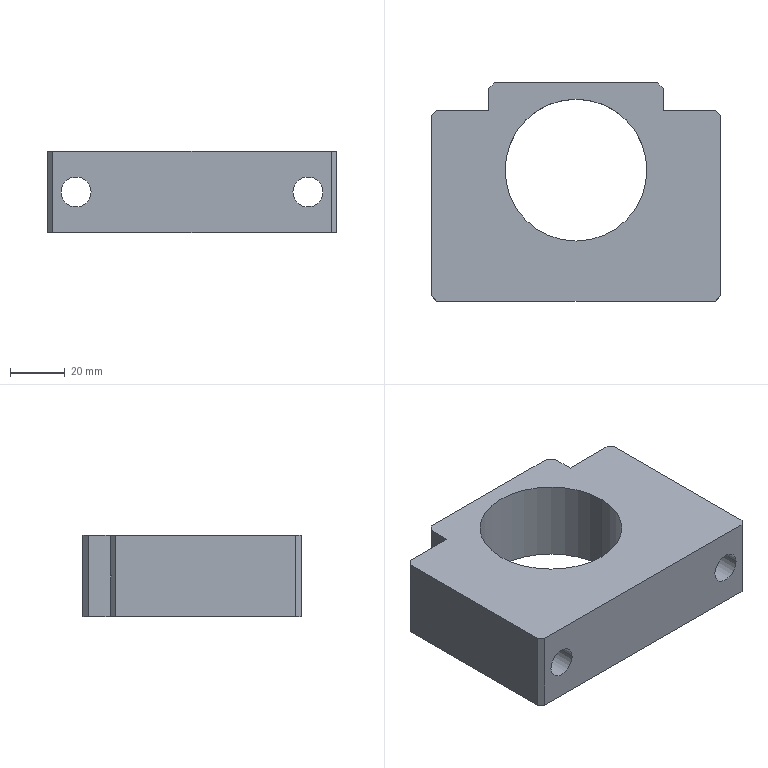Component | SolidWorks | BF_25_Part1-1 | 1 solid | 28 faces | box 106 x 80 x 30 mm | volume 161242 mm3 | plane 18 | cylinder 10 | commonest cylinder face diameters 11 x4 17.5 x4 52 x2
STEP:
#1=COLOUR_RGB('',0.7922,0.8196,0.9333);
#2=FILL_AREA_STYLE_COLOUR('',#1);
#3=FILL_AREA_STYLE('',(#2));
#4=SURFACE_STYLE_FILL_AREA(#3);
#5=SURFACE_SIDE_STYLE('',(#4));
#6=SURFACE_STYLE_USAGE(.BOTH.,#5);
#7=PRESENTATION_STYLE_ASSIGNMENT((#6));
#8=CARTESIAN_POINT('',(-0.7921,0.1356,-67.539));
#9=VERTEX_POINT('',#8);
#10=CARTESIAN_POINT('',(1.255,0.1356,-67.539));
#11=VERTEX_POINT('',#10);
#12=CARTESIAN_POINT('',(0.2315,0.1356,-67.539));
#13=DIRECTION('',(0.,0.,1.));
#14=DIRECTION('',(1.,0.,0.));
#15=AXIS2_PLACEMENT_3D('',#12,#13,#14);
#16=CIRCLE('',#15,1.024);
#17=EDGE_CURVE('',#9,#11,#16,.T.);
#18=ORIENTED_EDGE('',*,*,#17,.F.);
#19=CARTESIAN_POINT('',(-0.7921,0.1356,-66.358));
#20=VERTEX_POINT('',#19);
#21=CARTESIAN_POINT('',(-0.7921,0.1356,-67.539));
#22=DIRECTION('',(0.,0.,1.));
#23=VECTOR('',#22,39.37);
#24=LINE('',#21,#23);
#25=EDGE_CURVE('',#9,#20,#24,.T.);
#26=ORIENTED_EDGE('',*,*,#25,.T.);
#27=CARTESIAN_POINT('',(1.255,0.1356,-66.358));
#28=VERTEX_POINT('',#27);
#29=CARTESIAN_POINT('',(0.2315,0.1356,-66.358));
#30=DIRECTION('',(0.,0.,1.));
#31=DIRECTION('',(1.,0.,0.));
#32=AXIS2_PLACEMENT_3D('',#29,#30,#31);
#33=CIRCLE('',#32,1.024);
#34=EDGE_CURVE('',#20,#28,#33,.T.);
#35=ORIENTED_EDGE('',*,*,#34,.T.);
#36=CARTESIAN_POINT('',(1.255,0.1356,-67.539));
#37=DIRECTION('',(0.,0.,1.));
#38=VECTOR('',#37,39.37);
#39=LINE('',#36,#38);
#40=EDGE_CURVE('',#11,#28,#39,.T.);
#41=ORIENTED_EDGE('',*,*,#40,.F.);
#42=EDGE_LOOP('',(#18,#26,#35,#41));
#43=FACE_OUTER_BOUND('',#42,.T.);
#44=CARTESIAN_POINT('',(0.2315,0.1356,-67.539));
#45=DIRECTION('',(0.,0.,1.));
#46=DIRECTION('',(1.,0.,0.));
#47=AXIS2_PLACEMENT_3D('',#44,#45,#46);
#48=CYLINDRICAL_SURFACE('',#47,1.024);
#49=ADVANCED_FACE('',(#43),#48,.F.);
#50=CARTESIAN_POINT('',(-1.225,-1.754,-66.949));
#51=VERTEX_POINT('',#50);
#52=CARTESIAN_POINT('',(-1.658,-1.754,-66.949));
#53=VERTEX_POINT('',#52);
#54=CARTESIAN_POINT('',(-1.442,-1.754,-66.949));
#55=DIRECTION('',(0.,1.,0.));
#56=DIRECTION('',(-1.,0.,0.));
#57=AXIS2_PLACEMENT_3D('',#54,#55,#56);
#58=CIRCLE('',#57,0.2165);
#59=EDGE_CURVE('',#51,#53,#58,.T.);
#60=ORIENTED_EDGE('',*,*,#59,.F.);
#61=CARTESIAN_POINT('',(-1.225,0.5687,-66.949));
#62=VERTEX_POINT('',#61);
#63=CARTESIAN_POINT('',(-1.225,-1.754,-66.949));
#64=DIRECTION('',(0.,1.,0.));
#65=VECTOR('',#64,39.37);
#66=LINE('',#63,#65);
#67=EDGE_CURVE('',#51,#62,#66,.T.);
#68=ORIENTED_EDGE('',*,*,#67,.T.);
#69=CARTESIAN_POINT('',(-1.658,0.5687,-66.949));
#70=VERTEX_POINT('',#69);
#71=CARTESIAN_POINT('',(-1.442,0.5687,-66.949));
#72=DIRECTION('',(0.,1.,0.));
#73=DIRECTION('',(-1.,0.,0.));
#74=AXIS2_PLACEMENT_3D('',#71,#72,#73);
#75=CIRCLE('',#74,0.2165);
#76=EDGE_CURVE('',#62,#70,#75,.T.);
#77=ORIENTED_EDGE('',*,*,#76,.T.);
#78=CARTESIAN_POINT('',(-1.658,-1.754,-66.949));
#79=DIRECTION('',(0.,1.,0.));
#80=VECTOR('',#79,39.37);
#81=LINE('',#78,#80);
#82=EDGE_CURVE('',#53,#70,#81,.T.);
#83=ORIENTED_EDGE('',*,*,#82,.F.);
#84=EDGE_LOOP('',(#60,#68,#77,#83));
#85=FACE_OUTER_BOUND('',#84,.T.);
#86=CARTESIAN_POINT('',(-1.442,-1.754,-66.949));
#87=DIRECTION('',(0.,1.,0.));
#88=DIRECTION('',(-1.,0.,0.));
#89=AXIS2_PLACEMENT_3D('',#86,#87,#88);
#90=CYLINDRICAL_SURFACE('',#89,0.2165);
#91=ADVANCED_FACE('',(#85),#90,.F.);
#92=CARTESIAN_POINT('',(-1.097,0.5687,-66.949));
#93=VERTEX_POINT('',#92);
#94=CARTESIAN_POINT('',(-1.786,0.5687,-66.949));
#95=VERTEX_POINT('',#94);
#96=CARTESIAN_POINT('',(-1.442,0.5687,-66.949));
#97=DIRECTION('',(0.,1.,0.));
#98=DIRECTION('',(-1.,0.,0.));
#99=AXIS2_PLACEMENT_3D('',#96,#97,#98);
#100=CIRCLE('',#99,0.3445);
#101=EDGE_CURVE('',#93,#95,#100,.T.);
#102=ORIENTED_EDGE('',*,*,#101,.F.);
#103=CARTESIAN_POINT('',(-1.097,1.002,-66.949));
#104=VERTEX_POINT('',#103);
#105=CARTESIAN_POINT('',(-1.097,-1.754,-66.949));
#106=DIRECTION('',(0.,1.,0.));
#107=VECTOR('',#106,39.37);
#108=LINE('',#105,#107);
#109=EDGE_CURVE('',#93,#104,#108,.T.);
#110=ORIENTED_EDGE('',*,*,#109,.T.);
#111=CARTESIAN_POINT('',(-1.779,1.002,-67.016));
#112=VERTEX_POINT('',#111);
#113=CARTESIAN_POINT('',(-1.442,1.002,-66.949));
#114=DIRECTION('',(0.,1.,0.));
#115=DIRECTION('',(0.,0.,1.));
#116=AXIS2_PLACEMENT_3D('',#113,#114,#115);
#117=CIRCLE('',#116,0.3445);
#118=EDGE_CURVE('',#104,#112,#117,.T.);
#119=ORIENTED_EDGE('',*,*,#118,.T.);
#120=CARTESIAN_POINT('',(-1.786,0.9951,-66.949));
#121=VERTEX_POINT('',#120);
#122=CARTESIAN_POINT('',(-1.779,1.002,-67.016));
#123=CARTESIAN_POINT('',(-1.784,0.9973,-66.994));
#124=CARTESIAN_POINT('',(-1.786,0.9951,-66.972));
#125=CARTESIAN_POINT('',(-1.786,0.9951,-66.949));
#126=(BOUNDED_CURVE()B_SPLINE_CURVE(3,(#122,#123,#124,#125),.UNSPECIFIED.,.F.,.F.)B_SPLINE_CURVE_WITH_KNOTS((4,4),(2.944,3.142),.UNSPECIFIED.)CURVE()GEOMETRIC_REPRESENTATION_ITEM()RATIONAL_B_SPLINE_CURVE((1.,0.9968,0.9968,1.))REPRESENTATION_ITEM(''));
#127=EDGE_CURVE('',#112,#121,#126,.T.);
#128=ORIENTED_EDGE('',*,*,#127,.T.);
#129=CARTESIAN_POINT('',(-1.786,-1.754,-66.949));
#130=DIRECTION('',(0.,1.,0.));
#131=VECTOR('',#130,39.37);
#132=LINE('',#129,#131);
#133=EDGE_CURVE('',#95,#121,#132,.T.);
#134=ORIENTED_EDGE('',*,*,#133,.F.);
#135=EDGE_LOOP('',(#102,#110,#119,#128,#134));
#136=FACE_OUTER_BOUND('',#135,.T.);
#137=CARTESIAN_POINT('',(-1.442,-1.754,-66.949));
#138=DIRECTION('',(0.,1.,0.));
#139=DIRECTION('',(-1.,0.,0.));
#140=AXIS2_PLACEMENT_3D('',#137,#138,#139);
#141=CYLINDRICAL_SURFACE('',#140,0.3445);
#142=ADVANCED_FACE('',(#136),#141,.F.);
#143=CARTESIAN_POINT('',(2.121,-1.754,-66.949));
#144=VERTEX_POINT('',#143);
#145=CARTESIAN_POINT('',(1.688,-1.754,-66.949));
#146=VERTEX_POINT('',#145);
#147=CARTESIAN_POINT('',(1.905,-1.754,-66.949));
#148=DIRECTION('',(0.,1.,0.));
#149=DIRECTION('',(-1.,0.,0.));
#150=AXIS2_PLACEMENT_3D('',#147,#148,#149);
#151=CIRCLE('',#150,0.2165);
#152=EDGE_CURVE('',#144,#146,#151,.T.);
#153=ORIENTED_EDGE('',*,*,#152,.F.);
#154=CARTESIAN_POINT('',(2.121,0.5687,-66.949));
#155=VERTEX_POINT('',#154);
#156=CARTESIAN_POINT('',(2.121,-1.754,-66.949));
#157=DIRECTION('',(0.,1.,0.));
#158=VECTOR('',#157,39.37);
#159=LINE('',#156,#158);
#160=EDGE_CURVE('',#144,#155,#159,.T.);
#161=ORIENTED_EDGE('',*,*,#160,.T.);
#162=CARTESIAN_POINT('',(1.688,0.5687,-66.949));
#163=VERTEX_POINT('',#162);
#164=CARTESIAN_POINT('',(1.905,0.5687,-66.949));
#165=DIRECTION('',(0.,1.,0.));
#166=DIRECTION('',(-1.,0.,0.));
#167=AXIS2_PLACEMENT_3D('',#164,#165,#166);
#168=CIRCLE('',#167,0.2165);
#169=EDGE_CURVE('',#155,#163,#168,.T.);
#170=ORIENTED_EDGE('',*,*,#169,.T.);
#171=CARTESIAN_POINT('',(1.688,-1.754,-66.949));
#172=DIRECTION('',(0.,1.,0.));
#173=VECTOR('',#172,39.37);
#174=LINE('',#171,#173);
#175=EDGE_CURVE('',#146,#163,#174,.T.);
#176=ORIENTED_EDGE('',*,*,#175,.F.);
#177=EDGE_LOOP('',(#153,#161,#170,#176));
#178=FACE_OUTER_BOUND('',#177,.T.);
#179=CARTESIAN_POINT('',(1.905,-1.754,-66.949));
#180=DIRECTION('',(0.,1.,0.));
#181=DIRECTION('',(-1.,0.,0.));
#182=AXIS2_PLACEMENT_3D('',#179,#180,#181);
#183=CYLINDRICAL_SURFACE('',#182,0.2165);
#184=ADVANCED_FACE('',(#178),#183,.F.);
#185=CARTESIAN_POINT('',(2.249,0.5687,-66.949));
#186=VERTEX_POINT('',#185);
#187=CARTESIAN_POINT('',(1.56,0.5687,-66.949));
#188=VERTEX_POINT('',#187);
#189=CARTESIAN_POINT('',(1.905,0.5687,-66.949));
#190=DIRECTION('',(0.,1.,0.));
#191=DIRECTION('',(-1.,0.,0.));
#192=AXIS2_PLACEMENT_3D('',#189,#190,#191);
#193=CIRCLE('',#192,0.3445);
#194=EDGE_CURVE('',#186,#188,#193,.T.);
#195=ORIENTED_EDGE('',*,*,#194,.F.);
#196=CARTESIAN_POINT('',(2.249,0.9951,-66.949));
#197=VERTEX_POINT('',#196);
#198=CARTESIAN_POINT('',(2.249,-1.754,-66.949));
#199=DIRECTION('',(0.,1.,0.));
#200=VECTOR('',#199,39.37);
#201=LINE('',#198,#200);
#202=EDGE_CURVE('',#186,#197,#201,.T.);
#203=ORIENTED_EDGE('',*,*,#202,.T.);
#204=CARTESIAN_POINT('',(2.243,1.002,-67.016));
#205=VERTEX_POINT('',#204);
#206=CARTESIAN_POINT('',(2.249,0.9951,-66.949));
#207=CARTESIAN_POINT('',(2.249,0.9951,-66.972));
#208=CARTESIAN_POINT('',(2.247,0.9973,-66.994));
#209=CARTESIAN_POINT('',(2.243,1.002,-67.016));
#210=(BOUNDED_CURVE()B_SPLINE_CURVE(3,(#206,#207,#208,#209),.UNSPECIFIED.,.F.,.F.)B_SPLINE_CURVE_WITH_KNOTS((4,4),(3.142,3.339),.UNSPECIFIED.)CURVE()GEOMETRIC_REPRESENTATION_ITEM()RATIONAL_B_SPLINE_CURVE((1.,0.9968,0.9968,1.))REPRESENTATION_ITEM(''));
#211=EDGE_CURVE('',#197,#205,#210,.T.);
#212=ORIENTED_EDGE('',*,*,#211,.T.);
#213=CARTESIAN_POINT('',(1.56,1.002,-66.949));
#214=VERTEX_POINT('',#213);
#215=CARTESIAN_POINT('',(1.905,1.002,-66.949));
#216=DIRECTION('',(0.,1.,0.));
#217=DIRECTION('',(0.,0.,1.));
#218=AXIS2_PLACEMENT_3D('',#215,#216,#217);
#219=CIRCLE('',#218,0.3445);
#220=EDGE_CURVE('',#205,#214,#219,.T.);
#221=ORIENTED_EDGE('',*,*,#220,.T.);
#222=CARTESIAN_POINT('',(1.56,-1.754,-66.949));
#223=DIRECTION('',(0.,1.,0.));
#224=VECTOR('',#223,39.37);
#225=LINE('',#222,#224);
#226=EDGE_CURVE('',#188,#214,#225,.T.);
#227=ORIENTED_EDGE('',*,*,#226,.F.);
#228=EDGE_LOOP('',(#195,#203,#212,#221,#227));
#229=FACE_OUTER_BOUND('',#228,.T.);
#230=CARTESIAN_POINT('',(1.905,-1.754,-66.949));
#231=DIRECTION('',(0.,1.,0.));
#232=DIRECTION('',(-1.,0.,0.));
#233=AXIS2_PLACEMENT_3D('',#230,#231,#232);
#234=CYLINDRICAL_SURFACE('',#233,0.3445);
#235=ADVANCED_FACE('',(#229),#234,.F.);
#236=ORIENTED_EDGE('',*,*,#127,.F.);
#237=CARTESIAN_POINT('',(-1.779,1.002,-67.539));
#238=VERTEX_POINT('',#237);
#239=CARTESIAN_POINT('',(-1.779,1.002,-67.539));
#240=DIRECTION('',(0.,0.,1.));
#241=VECTOR('',#240,39.37);
#242=LINE('',#239,#241);
#243=EDGE_CURVE('',#238,#112,#242,.T.);
#244=ORIENTED_EDGE('',*,*,#243,.F.);
#245=CARTESIAN_POINT('',(-1.855,0.9262,-67.539));
#246=VERTEX_POINT('',#245);
#247=CARTESIAN_POINT('',(-1.779,1.002,-67.539));
#248=DIRECTION('',(-0.7071,-0.7071,0.));
#249=VECTOR('',#248,39.37);
#250=LINE('',#247,#249);
#251=EDGE_CURVE('',#238,#246,#250,.T.);
#252=ORIENTED_EDGE('',*,*,#251,.T.);
#253=CARTESIAN_POINT('',(-1.855,0.9262,-66.358));
#254=VERTEX_POINT('',#253);
#255=CARTESIAN_POINT('',(-1.855,0.9262,-67.539));
#256=DIRECTION('',(0.,0.,1.));
#257=VECTOR('',#256,39.37);
#258=LINE('',#255,#257);
#259=EDGE_CURVE('',#246,#254,#258,.T.);
#260=ORIENTED_EDGE('',*,*,#259,.T.);
#261=CARTESIAN_POINT('',(-1.779,1.002,-66.358));
#262=VERTEX_POINT('',#261);
#263=CARTESIAN_POINT('',(-1.779,1.002,-66.358));
#264=DIRECTION('',(-0.7071,-0.7071,0.));
#265=VECTOR('',#264,39.37);
#266=LINE('',#263,#265);
#267=EDGE_CURVE('',#262,#254,#266,.T.);
#268=ORIENTED_EDGE('',*,*,#267,.F.);
#269=CARTESIAN_POINT('',(-1.779,1.002,-66.881));
#270=VERTEX_POINT('',#269);
#271=CARTESIAN_POINT('',(-1.779,1.002,-67.539));
#272=DIRECTION('',(0.,0.,1.));
#273=VECTOR('',#272,39.37);
#274=LINE('',#271,#273);
#275=EDGE_CURVE('',#270,#262,#274,.T.);
#276=ORIENTED_EDGE('',*,*,#275,.F.);
#277=CARTESIAN_POINT('',(-1.786,0.9951,-66.949));
#278=CARTESIAN_POINT('',(-1.786,0.9951,-66.926));
#279=CARTESIAN_POINT('',(-1.784,0.9973,-66.904));
#280=CARTESIAN_POINT('',(-1.779,1.002,-66.881));
#281=(BOUNDED_CURVE()B_SPLINE_CURVE(3,(#277,#278,#279,#280),.UNSPECIFIED.,.F.,.F.)B_SPLINE_CURVE_WITH_KNOTS((4,4),(3.142,3.339),.UNSPECIFIED.)CURVE()GEOMETRIC_REPRESENTATION_ITEM()RATIONAL_B_SPLINE_CURVE((1.,0.9968,0.9968,1.))REPRESENTATION_ITEM(''));
#282=EDGE_CURVE('',#121,#270,#281,.T.);
#283=ORIENTED_EDGE('',*,*,#282,.F.);
#284=EDGE_LOOP('',(#236,#244,#252,#260,#268,#276,#283));
#285=FACE_OUTER_BOUND('',#284,.T.);
#286=CARTESIAN_POINT('',(-1.779,1.002,-67.539));
#287=DIRECTION('',(-0.7071,0.7071,0.));
#288=DIRECTION('',(-0.7071,-0.7071,0.));
#289=AXIS2_PLACEMENT_3D('',#286,#287,#288);
#290=PLANE('',#289);
#291=ADVANCED_FACE('',(#285),#290,.T.);
#292=CARTESIAN_POINT('',(-1.855,-1.679,-66.358));
#293=VERTEX_POINT('',#292);
#294=CARTESIAN_POINT('',(-1.855,0.9262,-66.358));
#295=DIRECTION('',(0.,-1.,0.));
#296=VECTOR('',#295,39.37);
#297=LINE('',#294,#296);
#298=EDGE_CURVE('',#254,#293,#297,.T.);
#299=ORIENTED_EDGE('',*,*,#298,.F.);
#300=ORIENTED_EDGE('',*,*,#259,.F.);
#301=CARTESIAN_POINT('',(-1.855,-1.679,-67.539));
#302=VERTEX_POINT('',#301);
#303=CARTESIAN_POINT('',(-1.855,0.9262,-67.539));
#304=DIRECTION('',(0.,-1.,0.));
#305=VECTOR('',#304,39.37);
#306=LINE('',#303,#305);
#307=EDGE_CURVE('',#246,#302,#306,.T.);
#308=ORIENTED_EDGE('',*,*,#307,.T.);
#309=CARTESIAN_POINT('',(-1.855,-1.679,-67.539));
#310=DIRECTION('',(0.,0.,1.));
#311=VECTOR('',#310,39.37);
#312=LINE('',#309,#311);
#313=EDGE_CURVE('',#302,#293,#312,.T.);
#314=ORIENTED_EDGE('',*,*,#313,.T.);
#315=EDGE_LOOP('',(#299,#300,#308,#314));
#316=FACE_OUTER_BOUND('',#315,.T.);
#317=CARTESIAN_POINT('',(-1.855,0.9262,-67.539));
#318=DIRECTION('',(-1.,0.,0.));
#319=DIRECTION('',(0.,0.,1.));
#320=AXIS2_PLACEMENT_3D('',#317,#318,#319);
#321=PLANE('',#320);
#322=ADVANCED_FACE('',(#316),#321,.T.);
#323=CARTESIAN_POINT('',(-1.779,-1.754,-66.358));
#324=VERTEX_POINT('',#323);
#325=CARTESIAN_POINT('',(-1.855,-1.679,-66.358));
#326=DIRECTION('',(0.7071,-0.7071,0.));
#327=VECTOR('',#326,39.37);
#328=LINE('',#325,#327);
#329=EDGE_CURVE('',#293,#324,#328,.T.);
#330=ORIENTED_EDGE('',*,*,#329,.F.);
#331=ORIENTED_EDGE('',*,*,#313,.F.);
#332=CARTESIAN_POINT('',(-1.779,-1.754,-67.539));
#333=VERTEX_POINT('',#332);
#334=CARTESIAN_POINT('',(-1.855,-1.679,-67.539));
#335=DIRECTION('',(0.7071,-0.7071,0.));
#336=VECTOR('',#335,39.37);
#337=LINE('',#334,#336);
#338=EDGE_CURVE('',#302,#333,#337,.T.);
#339=ORIENTED_EDGE('',*,*,#338,.T.);
#340=CARTESIAN_POINT('',(-1.779,-1.754,-67.539));
#341=DIRECTION('',(0.,0.,1.));
#342=VECTOR('',#341,39.37);
#343=LINE('',#340,#342);
#344=EDGE_CURVE('',#333,#324,#343,.T.);
#345=ORIENTED_EDGE('',*,*,#344,.T.);
#346=EDGE_LOOP('',(#330,#331,#339,#345));
#347=FACE_OUTER_BOUND('',#346,.T.);
#348=CARTESIAN_POINT('',(-1.855,-1.679,-67.539));
#349=DIRECTION('',(-0.7071,-0.7071,0.));
#350=DIRECTION('',(0.7071,-0.7071,0.));
#351=AXIS2_PLACEMENT_3D('',#348,#349,#350);
#352=PLANE('',#351);
#353=ADVANCED_FACE('',(#347),#352,.T.);
#354=CARTESIAN_POINT('',(-1.442,-1.754,-66.949));
#355=DIRECTION('',(0.,1.,0.));
#356=DIRECTION('',(-1.,0.,0.));
#357=AXIS2_PLACEMENT_3D('',#354,#355,#356);
#358=CIRCLE('',#357,0.2165);
#359=EDGE_CURVE('',#53,#51,#358,.T.);
#360=ORIENTED_EDGE('',*,*,#359,.T.);
#361=ORIENTED_EDGE('',*,*,#59,.T.);
#362=EDGE_LOOP('',(#360,#361));
#363=FACE_BOUND('',#362,.T.);
#364=CARTESIAN_POINT('',(1.905,-1.754,-66.949));
#365=DIRECTION('',(0.,1.,0.));
#366=DIRECTION('',(-1.,0.,0.));
#367=AXIS2_PLACEMENT_3D('',#364,#365,#366);
#368=CIRCLE('',#367,0.2165);
#369=EDGE_CURVE('',#146,#144,#368,.T.);
#370=ORIENTED_EDGE('',*,*,#369,.T.);
#371=ORIENTED_EDGE('',*,*,#152,.T.);
#372=EDGE_LOOP('',(#370,#371));
#373=FACE_BOUND('',#372,.T.);
#374=CARTESIAN_POINT('',(2.243,-1.754,-66.358));
#375=VERTEX_POINT('',#374);
#376=CARTESIAN_POINT('',(-1.779,-1.754,-66.358));
#377=DIRECTION('',(1.,0.,0.));
#378=VECTOR('',#377,39.37);
#379=LINE('',#376,#378);
#380=EDGE_CURVE('',#324,#375,#379,.T.);
#381=ORIENTED_EDGE('',*,*,#380,.F.);
#382=ORIENTED_EDGE('',*,*,#344,.F.);
#383=CARTESIAN_POINT('',(2.243,-1.754,-67.539));
#384=VERTEX_POINT('',#383);
#385=CARTESIAN_POINT('',(-1.779,-1.754,-67.539));
#386=DIRECTION('',(1.,0.,0.));
#387=VECTOR('',#386,39.37);
#388=LINE('',#385,#387);
#389=EDGE_CURVE('',#333,#384,#388,.T.);
#390=ORIENTED_EDGE('',*,*,#389,.T.);
#391=CARTESIAN_POINT('',(2.243,-1.754,-67.539));
#392=DIRECTION('',(0.,0.,1.));
#393=VECTOR('',#392,39.37);
#394=LINE('',#391,#393);
#395=EDGE_CURVE('',#384,#375,#394,.T.);
#396=ORIENTED_EDGE('',*,*,#395,.T.);
#397=EDGE_LOOP('',(#381,#382,#390,#396));
#398=FACE_OUTER_BOUND('',#397,.T.);
#399=CARTESIAN_POINT('',(-1.779,-1.754,-67.539));
#400=DIRECTION('',(0.,-1.,0.));
#401=DIRECTION('',(0.,0.,-1.));
#402=AXIS2_PLACEMENT_3D('',#399,#400,#401);
#403=PLANE('',#402);
#404=ADVANCED_FACE('',(#363,#373,#398),#403,.T.);
#405=CARTESIAN_POINT('',(2.318,-1.679,-66.358));
#406=VERTEX_POINT('',#405);
#407=CARTESIAN_POINT('',(2.243,-1.754,-66.358));
#408=DIRECTION('',(0.7071,0.7071,0.));
#409=VECTOR('',#408,39.37);
#410=LINE('',#407,#409);
#411=EDGE_CURVE('',#375,#406,#410,.T.);
#412=ORIENTED_EDGE('',*,*,#411,.F.);
#413=ORIENTED_EDGE('',*,*,#395,.F.);
#414=CARTESIAN_POINT('',(2.318,-1.679,-67.539));
#415=VERTEX_POINT('',#414);
#416=CARTESIAN_POINT('',(2.243,-1.754,-67.539));
#417=DIRECTION('',(0.7071,0.7071,0.));
#418=VECTOR('',#417,39.37);
#419=LINE('',#416,#418);
#420=EDGE_CURVE('',#384,#415,#419,.T.);
#421=ORIENTED_EDGE('',*,*,#420,.T.);
#422=CARTESIAN_POINT('',(2.318,-1.679,-67.539));
#423=DIRECTION('',(0.,0.,1.));
#424=VECTOR('',#423,39.37);
#425=LINE('',#422,#424);
#426=EDGE_CURVE('',#415,#406,#425,.T.);
#427=ORIENTED_EDGE('',*,*,#426,.T.);
#428=EDGE_LOOP('',(#412,#413,#421,#427));
#429=FACE_OUTER_BOUND('',#428,.T.);
#430=CARTESIAN_POINT('',(2.243,-1.754,-67.539));
#431=DIRECTION('',(0.7071,-0.7071,0.));
#432=DIRECTION('',(0.7071,0.7071,0.));
#433=AXIS2_PLACEMENT_3D('',#430,#431,#432);
#434=PLANE('',#433);
#435=ADVANCED_FACE('',(#429),#434,.T.);
#436=CARTESIAN_POINT('',(2.318,0.9262,-66.358));
#437=VERTEX_POINT('',#436);
#438=CARTESIAN_POINT('',(2.318,-1.679,-66.358));
#439=DIRECTION('',(0.,1.,0.));
#440=VECTOR('',#439,39.37);
#441=LINE('',#438,#440);
#442=EDGE_CURVE('',#406,#437,#441,.T.);
#443=ORIENTED_EDGE('',*,*,#442,.F.);
#444=ORIENTED_EDGE('',*,*,#426,.F.);
#445=CARTESIAN_POINT('',(2.318,0.9262,-67.539));
#446=VERTEX_POINT('',#445);
#447=CARTESIAN_POINT('',(2.318,-1.679,-67.539));
#448=DIRECTION('',(0.,1.,0.));
#449=VECTOR('',#448,39.37);
#450=LINE('',#447,#449);
#451=EDGE_CURVE('',#415,#446,#450,.T.);
#452=ORIENTED_EDGE('',*,*,#451,.T.);
#453=CARTESIAN_POINT('',(2.318,0.9262,-67.539));
#454=DIRECTION('',(0.,0.,1.));
#455=VECTOR('',#454,39.37);
#456=LINE('',#453,#455);
#457=EDGE_CURVE('',#446,#437,#456,.T.);
#458=ORIENTED_EDGE('',*,*,#457,.T.);
#459=EDGE_LOOP('',(#443,#444,#452,#458));
#460=FACE_OUTER_BOUND('',#459,.T.);
#461=CARTESIAN_POINT('',(2.318,-1.679,-67.539));
#462=DIRECTION('',(1.,0.,0.));
#463=DIRECTION('',(0.,0.,-1.));
#464=AXIS2_PLACEMENT_3D('',#461,#462,#463);
#465=PLANE('',#464);
#466=ADVANCED_FACE('',(#460),#465,.T.);
#467=CARTESIAN_POINT('',(2.243,1.002,-66.881));
#468=VERTEX_POINT('',#467);
#469=CARTESIAN_POINT('',(2.243,1.002,-66.881));
#470=CARTESIAN_POINT('',(2.247,0.9973,-66.904));
#471=CARTESIAN_POINT('',(2.249,0.9951,-66.926));
#472=CARTESIAN_POINT('',(2.249,0.9951,-66.949));
#473=(BOUNDED_CURVE()B_SPLINE_CURVE(3,(#469,#470,#471,#472),.UNSPECIFIED.,.F.,.F.)B_SPLINE_CURVE_WITH_KNOTS((4,4),(2.944,3.142),.UNSPECIFIED.)CURVE()GEOMETRIC_REPRESENTATION_ITEM()RATIONAL_B_SPLINE_CURVE((1.,0.9968,0.9968,1.))REPRESENTATION_ITEM(''));
#474=EDGE_CURVE('',#468,#197,#473,.T.);
#475=ORIENTED_EDGE('',*,*,#474,.F.);
#476=CARTESIAN_POINT('',(2.243,1.002,-66.358));
#477=VERTEX_POINT('',#476);
#478=CARTESIAN_POINT('',(2.243,1.002,-67.539));
#479=DIRECTION('',(0.,0.,1.));
#480=VECTOR('',#479,39.37);
#481=LINE('',#478,#480);
#482=EDGE_CURVE('',#468,#477,#481,.T.);
#483=ORIENTED_EDGE('',*,*,#482,.T.);
#484=CARTESIAN_POINT('',(2.318,0.9262,-66.358));
#485=DIRECTION('',(-0.7071,0.7071,0.));
#486=VECTOR('',#485,39.37);
#487=LINE('',#484,#486);
#488=EDGE_CURVE('',#437,#477,#487,.T.);
#489=ORIENTED_EDGE('',*,*,#488,.F.);
#490=ORIENTED_EDGE('',*,*,#457,.F.);
#491=CARTESIAN_POINT('',(2.243,1.002,-67.539));
#492=VERTEX_POINT('',#491);
#493=CARTESIAN_POINT('',(2.318,0.9262,-67.539));
#494=DIRECTION('',(-0.7071,0.7071,0.));
#495=VECTOR('',#494,39.37);
#496=LINE('',#493,#495);
#497=EDGE_CURVE('',#446,#492,#496,.T.);
#498=ORIENTED_EDGE('',*,*,#497,.T.);
#499=CARTESIAN_POINT('',(2.243,1.002,-67.539));
#500=DIRECTION('',(0.,0.,1.));
#501=VECTOR('',#500,39.37);
#502=LINE('',#499,#501);
#503=EDGE_CURVE('',#492,#205,#502,.T.);
#504=ORIENTED_EDGE('',*,*,#503,.T.);
#505=ORIENTED_EDGE('',*,*,#211,.F.);
#506=EDGE_LOOP('',(#475,#483,#489,#490,#498,#504,#505));
#507=FACE_OUTER_BOUND('',#506,.T.);
#508=CARTESIAN_POINT('',(2.318,0.9262,-67.539));
#509=DIRECTION('',(0.7071,0.7071,0.));
#510=DIRECTION('',(-0.7071,0.7071,0.));
#511=AXIS2_PLACEMENT_3D('',#508,#509,#510);
#512=PLANE('',#511);
#513=ADVANCED_FACE('',(#507),#512,.T.);
#514=ORIENTED_EDGE('',*,*,#482,.F.);
#515=CARTESIAN_POINT('',(1.905,1.002,-66.949));
#516=DIRECTION('',(0.,1.,0.));
#517=DIRECTION('',(0.,0.,1.));
#518=AXIS2_PLACEMENT_3D('',#515,#516,#517);
#519=CIRCLE('',#518,0.3445);
#520=EDGE_CURVE('',#214,#468,#519,.T.);
#521=ORIENTED_EDGE('',*,*,#520,.F.);
#522=ORIENTED_EDGE('',*,*,#220,.F.);
#523=ORIENTED_EDGE('',*,*,#503,.F.);
#524=CARTESIAN_POINT('',(1.491,1.002,-67.539));
#525=VERTEX_POINT('',#524);
#526=CARTESIAN_POINT('',(2.243,1.002,-67.539));
#527=DIRECTION('',(-1.,0.,0.));
#528=VECTOR('',#527,39.37);
#529=LINE('',#526,#528);
#530=EDGE_CURVE('',#492,#525,#529,.T.);
#531=ORIENTED_EDGE('',*,*,#530,.T.);
#532=CARTESIAN_POINT('',(1.491,1.002,-66.358));
#533=VERTEX_POINT('',#532);
#534=CARTESIAN_POINT('',(1.491,1.002,-67.539));
#535=DIRECTION('',(0.,0.,1.));
#536=VECTOR('',#535,39.37);
#537=LINE('',#534,#536);
#538=EDGE_CURVE('',#525,#533,#537,.T.);
#539=ORIENTED_EDGE('',*,*,#538,.T.);
#540=CARTESIAN_POINT('',(2.243,1.002,-66.358));
#541=DIRECTION('',(-1.,0.,0.));
#542=VECTOR('',#541,39.37);
#543=LINE('',#540,#542);
#544=EDGE_CURVE('',#477,#533,#543,.T.);
#545=ORIENTED_EDGE('',*,*,#544,.F.);
#546=EDGE_LOOP('',(#514,#521,#522,#523,#531,#539,#545));
#547=FACE_OUTER_BOUND('',#546,.T.);
#548=CARTESIAN_POINT('',(2.243,1.002,-67.539));
#549=DIRECTION('',(0.,1.,0.));
#550=DIRECTION('',(0.,0.,1.));
#551=AXIS2_PLACEMENT_3D('',#548,#549,#550);
#552=PLANE('',#551);
#553=ADVANCED_FACE('',(#547),#552,.T.);
#554=CARTESIAN_POINT('',(1.491,1.317,-66.358));
#555=VERTEX_POINT('',#554);
#556=CARTESIAN_POINT('',(1.491,1.002,-66.358));
#557=DIRECTION('',(0.,1.,0.));
#558=VECTOR('',#557,39.37);
#559=LINE('',#556,#558);
#560=EDGE_CURVE('',#533,#555,#559,.T.);
#561=ORIENTED_EDGE('',*,*,#560,.F.);
#562=ORIENTED_EDGE('',*,*,#538,.F.);
#563=CARTESIAN_POINT('',(1.491,1.317,-67.539));
#564=VERTEX_POINT('',#563);
#565=CARTESIAN_POINT('',(1.491,1.002,-67.539));
#566=DIRECTION('',(0.,1.,0.));
#567=VECTOR('',#566,39.37);
#568=LINE('',#565,#567);
#569=EDGE_CURVE('',#525,#564,#568,.T.);
#570=ORIENTED_EDGE('',*,*,#569,.T.);
#571=CARTESIAN_POINT('',(1.491,1.317,-67.539));
#572=DIRECTION('',(0.,0.,1.));
#573=VECTOR('',#572,39.37);
#574=LINE('',#571,#573);
#575=EDGE_CURVE('',#564,#555,#574,.T.);
#576=ORIENTED_EDGE('',*,*,#575,.T.);
#577=EDGE_LOOP('',(#561,#562,#570,#576));
#578=FACE_OUTER_BOUND('',#577,.T.);
#579=CARTESIAN_POINT('',(1.491,1.002,-67.539));
#580=DIRECTION('',(1.,0.,0.));
#581=DIRECTION('',(0.,0.,-1.));
#582=AXIS2_PLACEMENT_3D('',#579,#580,#581);
#583=PLANE('',#582);
#584=ADVANCED_FACE('',(#578),#583,.T.);
#585=CARTESIAN_POINT('',(1.413,1.395,-66.358));
#586=VERTEX_POINT('',#585);
#587=CARTESIAN_POINT('',(1.491,1.317,-66.358));
#588=DIRECTION('',(-0.7071,0.7071,0.));
#589=VECTOR('',#588,39.37);
#590=LINE('',#587,#589);
#591=EDGE_CURVE('',#555,#586,#590,.T.);
#592=ORIENTED_EDGE('',*,*,#591,.F.);
#593=ORIENTED_EDGE('',*,*,#575,.F.);
#594=CARTESIAN_POINT('',(1.413,1.395,-67.539));
#595=VERTEX_POINT('',#594);
#596=CARTESIAN_POINT('',(1.491,1.317,-67.539));
#597=DIRECTION('',(-0.7071,0.7071,0.));
#598=VECTOR('',#597,39.37);
#599=LINE('',#596,#598);
#600=EDGE_CURVE('',#564,#595,#599,.T.);
#601=ORIENTED_EDGE('',*,*,#600,.T.);
#602=CARTESIAN_POINT('',(1.413,1.395,-67.539));
#603=DIRECTION('',(0.,0.,1.));
#604=VECTOR('',#603,39.37);
#605=LINE('',#602,#604);
#606=EDGE_CURVE('',#595,#586,#605,.T.);
#607=ORIENTED_EDGE('',*,*,#606,.T.);
#608=EDGE_LOOP('',(#592,#593,#601,#607));
#609=FACE_OUTER_BOUND('',#608,.T.);
#610=CARTESIAN_POINT('',(1.491,1.317,-67.539));
#611=DIRECTION('',(0.7071,0.7071,0.));
#612=DIRECTION('',(-0.7071,0.7071,0.));
#613=AXIS2_PLACEMENT_3D('',#610,#611,#612);
#614=PLANE('',#613);
#615=ADVANCED_FACE('',(#609),#614,.T.);
#616=CARTESIAN_POINT('',(-0.9496,1.395,-66.358));
#617=VERTEX_POINT('',#616);
#618=CARTESIAN_POINT('',(1.413,1.395,-66.358));
#619=DIRECTION('',(-1.,0.,0.));
#620=VECTOR('',#619,39.37);
#621=LINE('',#618,#620);
#622=EDGE_CURVE('',#586,#617,#621,.T.);
#623=ORIENTED_EDGE('',*,*,#622,.F.);
#624=ORIENTED_EDGE('',*,*,#606,.F.);
#625=CARTESIAN_POINT('',(-0.9496,1.395,-67.539));
#626=VERTEX_POINT('',#625);
#627=CARTESIAN_POINT('',(1.413,1.395,-67.539));
#628=DIRECTION('',(-1.,0.,0.));
#629=VECTOR('',#628,39.37);
#630=LINE('',#627,#629);
#631=EDGE_CURVE('',#595,#626,#630,.T.);
#632=ORIENTED_EDGE('',*,*,#631,.T.);
#633=CARTESIAN_POINT('',(-0.9496,1.395,-67.539));
#634=DIRECTION('',(0.,0.,1.));
#635=VECTOR('',#634,39.37);
#636=LINE('',#633,#635);
#637=EDGE_CURVE('',#626,#617,#636,.T.);
#638=ORIENTED_EDGE('',*,*,#637,.T.);
#639=EDGE_LOOP('',(#623,#624,#632,#638));
#640=FACE_OUTER_BOUND('',#639,.T.);
#641=CARTESIAN_POINT('',(1.413,1.395,-67.539));
#642=DIRECTION('',(0.,1.,0.));
#643=DIRECTION('',(0.,0.,1.));
#644=AXIS2_PLACEMENT_3D('',#641,#642,#643);
#645=PLANE('',#644);
#646=ADVANCED_FACE('',(#640),#645,.T.);
#647=CARTESIAN_POINT('',(-1.028,1.317,-66.358));
#648=VERTEX_POINT('',#647);
#649=CARTESIAN_POINT('',(-0.9496,1.395,-66.358));
#650=DIRECTION('',(-0.7071,-0.7071,0.));
#651=VECTOR('',#650,39.37);
#652=LINE('',#649,#651);
#653=EDGE_CURVE('',#617,#648,#652,.T.);
#654=ORIENTED_EDGE('',*,*,#653,.F.);
#655=ORIENTED_EDGE('',*,*,#637,.F.);
#656=CARTESIAN_POINT('',(-1.028,1.317,-67.539));
#657=VERTEX_POINT('',#656);
#658=CARTESIAN_POINT('',(-0.9496,1.395,-67.539));
#659=DIRECTION('',(-0.7071,-0.7071,0.));
#660=VECTOR('',#659,39.37);
#661=LINE('',#658,#660);
#662=EDGE_CURVE('',#626,#657,#661,.T.);
#663=ORIENTED_EDGE('',*,*,#662,.T.);
#664=CARTESIAN_POINT('',(-1.028,1.317,-67.539));
#665=DIRECTION('',(0.,0.,1.));
#666=VECTOR('',#665,39.37);
#667=LINE('',#664,#666);
#668=EDGE_CURVE('',#657,#648,#667,.T.);
#669=ORIENTED_EDGE('',*,*,#668,.T.);
#670=EDGE_LOOP('',(#654,#655,#663,#669));
#671=FACE_OUTER_BOUND('',#670,.T.);
#672=CARTESIAN_POINT('',(-0.9496,1.395,-67.539));
#673=DIRECTION('',(-0.7071,0.7071,0.));
#674=DIRECTION('',(-0.7071,-0.7071,0.));
#675=AXIS2_PLACEMENT_3D('',#672,#673,#674);
#676=PLANE('',#675);
#677=ADVANCED_FACE('',(#671),#676,.T.);
#678=CARTESIAN_POINT('',(-1.028,1.002,-66.358));
#679=VERTEX_POINT('',#678);
#680=CARTESIAN_POINT('',(-1.028,1.317,-66.358));
#681=DIRECTION('',(0.,-1.,0.));
#682=VECTOR('',#681,39.37);
#683=LINE('',#680,#682);
#684=EDGE_CURVE('',#648,#679,#683,.T.);
#685=ORIENTED_EDGE('',*,*,#684,.F.);
#686=ORIENTED_EDGE('',*,*,#668,.F.);
#687=CARTESIAN_POINT('',(-1.028,1.002,-67.539));
#688=VERTEX_POINT('',#687);
#689=CARTESIAN_POINT('',(-1.028,1.317,-67.539));
#690=DIRECTION('',(0.,-1.,0.));
#691=VECTOR('',#690,39.37);
#692=LINE('',#689,#691);
#693=EDGE_CURVE('',#657,#688,#692,.T.);
#694=ORIENTED_EDGE('',*,*,#693,.T.);
#695=CARTESIAN_POINT('',(-1.028,1.002,-67.539));
#696=DIRECTION('',(0.,0.,1.));
#697=VECTOR('',#696,39.37);
#698=LINE('',#695,#697);
#699=EDGE_CURVE('',#688,#679,#698,.T.);
#700=ORIENTED_EDGE('',*,*,#699,.T.);
#701=EDGE_LOOP('',(#685,#686,#694,#700));
#702=FACE_OUTER_BOUND('',#701,.T.);
#703=CARTESIAN_POINT('',(-1.028,1.317,-67.539));
#704=DIRECTION('',(-1.,0.,0.));
#705=DIRECTION('',(0.,0.,1.));
#706=AXIS2_PLACEMENT_3D('',#703,#704,#705);
#707=PLANE('',#706);
#708=ADVANCED_FACE('',(#702),#707,.T.);
#709=ORIENTED_EDGE('',*,*,#243,.T.);
#710=ORIENTED_EDGE('',*,*,#118,.F.);
#711=CARTESIAN_POINT('',(-1.442,1.002,-66.949));
#712=DIRECTION('',(0.,1.,0.));
#713=DIRECTION('',(0.,0.,1.));
#714=AXIS2_PLACEMENT_3D('',#711,#712,#713);
#715=CIRCLE('',#714,0.3445);
#716=EDGE_CURVE('',#270,#104,#715,.T.);
#717=ORIENTED_EDGE('',*,*,#716,.F.);
#718=ORIENTED_EDGE('',*,*,#275,.T.);
#719=CARTESIAN_POINT('',(-1.028,1.002,-66.358));
#720=DIRECTION('',(-1.,0.,0.));
#721=VECTOR('',#720,39.37);
#722=LINE('',#719,#721);
#723=EDGE_CURVE('',#679,#262,#722,.T.);
#724=ORIENTED_EDGE('',*,*,#723,.F.);
#725=ORIENTED_EDGE('',*,*,#699,.F.);
#726=CARTESIAN_POINT('',(-1.028,1.002,-67.539));
#727=DIRECTION('',(-1.,0.,0.));
#728=VECTOR('',#727,39.37);
#729=LINE('',#726,#728);
#730=EDGE_CURVE('',#688,#238,#729,.T.);
#731=ORIENTED_EDGE('',*,*,#730,.T.);
#732=EDGE_LOOP('',(#709,#710,#717,#718,#724,#725,#731));
#733=FACE_OUTER_BOUND('',#732,.T.);
#734=CARTESIAN_POINT('',(-1.028,1.002,-67.539));
#735=DIRECTION('',(0.,1.,0.));
#736=DIRECTION('',(0.,0.,1.));
#737=AXIS2_PLACEMENT_3D('',#734,#735,#736);
#738=PLANE('',#737);
#739=ADVANCED_FACE('',(#733),#738,.T.);
#740=CARTESIAN_POINT('',(0.2315,0.1356,-67.539));
#741=DIRECTION('',(0.,0.,1.));
#742=DIRECTION('',(1.,0.,0.));
#743=AXIS2_PLACEMENT_3D('',#740,#741,#742);
#744=CIRCLE('',#743,1.024);
#745=EDGE_CURVE('',#11,#9,#744,.T.);
#746=ORIENTED_EDGE('',*,*,#745,.T.);
#747=ORIENTED_EDGE('',*,*,#17,.T.);
#748=EDGE_LOOP('',(#746,#747));
#749=FACE_BOUND('',#748,.T.);
#750=ORIENTED_EDGE('',*,*,#251,.F.);
#751=ORIENTED_EDGE('',*,*,#730,.F.);
#752=ORIENTED_EDGE('',*,*,#693,.F.);
#753=ORIENTED_EDGE('',*,*,#662,.F.);
#754=ORIENTED_EDGE('',*,*,#631,.F.);
#755=ORIENTED_EDGE('',*,*,#600,.F.);
#756=ORIENTED_EDGE('',*,*,#569,.F.);
#757=ORIENTED_EDGE('',*,*,#530,.F.);
#758=ORIENTED_EDGE('',*,*,#497,.F.);
#759=ORIENTED_EDGE('',*,*,#451,.F.);
#760=ORIENTED_EDGE('',*,*,#420,.F.);
#761=ORIENTED_EDGE('',*,*,#389,.F.);
#762=ORIENTED_EDGE('',*,*,#338,.F.);
#763=ORIENTED_EDGE('',*,*,#307,.F.);
#764=EDGE_LOOP('',(#750,#751,#752,#753,#754,#755,#756,#757,#758,#759,#760,#761,#762,#763));
#765=FACE_OUTER_BOUND('',#764,.T.);
#766=CARTESIAN_POINT('',(0.01342,2.795,-67.539));
#767=DIRECTION('',(0.,0.,-1.));
#768=DIRECTION('',(-1.,0.,0.));
#769=AXIS2_PLACEMENT_3D('',#766,#767,#768);
#770=PLANE('',#769);
#771=ADVANCED_FACE('',(#749,#765),#770,.T.);
#772=CARTESIAN_POINT('',(0.2315,0.1356,-66.358));
#773=DIRECTION('',(0.,0.,1.));
#774=DIRECTION('',(1.,0.,0.));
#775=AXIS2_PLACEMENT_3D('',#772,#773,#774);
#776=CIRCLE('',#775,1.024);
#777=EDGE_CURVE('',#28,#20,#776,.T.);
#778=ORIENTED_EDGE('',*,*,#777,.F.);
#779=ORIENTED_EDGE('',*,*,#34,.F.);
#780=EDGE_LOOP('',(#778,#779));
#781=FACE_BOUND('',#780,.T.);
#782=ORIENTED_EDGE('',*,*,#267,.T.);
#783=ORIENTED_EDGE('',*,*,#298,.T.);
#784=ORIENTED_EDGE('',*,*,#329,.T.);
#785=ORIENTED_EDGE('',*,*,#380,.T.);
#786=ORIENTED_EDGE('',*,*,#411,.T.);
#787=ORIENTED_EDGE('',*,*,#442,.T.);
#788=ORIENTED_EDGE('',*,*,#488,.T.);
#789=ORIENTED_EDGE('',*,*,#544,.T.);
#790=ORIENTED_EDGE('',*,*,#560,.T.);
#791=ORIENTED_EDGE('',*,*,#591,.T.);
#792=ORIENTED_EDGE('',*,*,#622,.T.);
#793=ORIENTED_EDGE('',*,*,#653,.T.);
#794=ORIENTED_EDGE('',*,*,#684,.T.);
#795=ORIENTED_EDGE('',*,*,#723,.T.);
#796=EDGE_LOOP('',(#782,#783,#784,#785,#786,#787,#788,#789,#790,#791,#792,#793,#794,#795));
#797=FACE_OUTER_BOUND('',#796,.T.);
#798=CARTESIAN_POINT('',(0.01342,2.795,-66.358));
#799=DIRECTION('',(0.,0.,-1.));
#800=DIRECTION('',(-1.,0.,0.));
#801=AXIS2_PLACEMENT_3D('',#798,#799,#800);
#802=PLANE('',#801);
#803=ADVANCED_FACE('',(#781,#797),#802,.F.);
#804=ORIENTED_EDGE('',*,*,#202,.F.);
#805=CARTESIAN_POINT('',(1.905,0.5687,-66.949));
#806=DIRECTION('',(0.,1.,0.));
#807=DIRECTION('',(-1.,0.,0.));
#808=AXIS2_PLACEMENT_3D('',#805,#806,#807);
#809=CIRCLE('',#808,0.3445);
#810=EDGE_CURVE('',#188,#186,#809,.T.);
#811=ORIENTED_EDGE('',*,*,#810,.F.);
#812=ORIENTED_EDGE('',*,*,#226,.T.);
#813=ORIENTED_EDGE('',*,*,#520,.T.);
#814=ORIENTED_EDGE('',*,*,#474,.T.);
#815=EDGE_LOOP('',(#804,#811,#812,#813,#814));
#816=FACE_OUTER_BOUND('',#815,.T.);
#817=CARTESIAN_POINT('',(1.905,-1.754,-66.949));
#818=DIRECTION('',(0.,1.,0.));
#819=DIRECTION('',(-1.,0.,0.));
#820=AXIS2_PLACEMENT_3D('',#817,#818,#819);
#821=CYLINDRICAL_SURFACE('',#820,0.3445);
#822=ADVANCED_FACE('',(#816),#821,.F.);
#823=CARTESIAN_POINT('',(1.905,0.5687,-66.949));
#824=DIRECTION('',(0.,1.,0.));
#825=DIRECTION('',(-1.,0.,0.));
#826=AXIS2_PLACEMENT_3D('',#823,#824,#825);
#827=CIRCLE('',#826,0.2165);
#828=EDGE_CURVE('',#163,#155,#827,.T.);
#829=ORIENTED_EDGE('',*,*,#828,.F.);
#830=ORIENTED_EDGE('',*,*,#169,.F.);
#831=EDGE_LOOP('',(#829,#830));
#832=FACE_BOUND('',#831,.T.);
#833=ORIENTED_EDGE('',*,*,#810,.T.);
#834=ORIENTED_EDGE('',*,*,#194,.T.);
#835=EDGE_LOOP('',(#833,#834));
#836=FACE_OUTER_BOUND('',#835,.T.);
#837=CARTESIAN_POINT('',(1.905,0.5687,-67.293));
#838=DIRECTION('',(-0.,-1.,0.));
#839=DIRECTION('',(1.,-0.,0.));
#840=AXIS2_PLACEMENT_3D('',#837,#838,#839);
#841=PLANE('',#840);
#842=ADVANCED_FACE('',(#832,#836),#841,.F.);
#843=ORIENTED_EDGE('',*,*,#160,.F.);
#844=ORIENTED_EDGE('',*,*,#369,.F.);
#845=ORIENTED_EDGE('',*,*,#175,.T.);
#846=ORIENTED_EDGE('',*,*,#828,.T.);
#847=EDGE_LOOP('',(#843,#844,#845,#846));
#848=FACE_OUTER_BOUND('',#847,.T.);
#849=CARTESIAN_POINT('',(1.905,-1.754,-66.949));
#850=DIRECTION('',(0.,1.,0.));
#851=DIRECTION('',(-1.,0.,0.));
#852=AXIS2_PLACEMENT_3D('',#849,#850,#851);
#853=CYLINDRICAL_SURFACE('',#852,0.2165);
#854=ADVANCED_FACE('',(#848),#853,.F.);
#855=ORIENTED_EDGE('',*,*,#109,.F.);
#856=CARTESIAN_POINT('',(-1.442,0.5687,-66.949));
#857=DIRECTION('',(0.,1.,0.));
#858=DIRECTION('',(-1.,0.,0.));
#859=AXIS2_PLACEMENT_3D('',#856,#857,#858);
#860=CIRCLE('',#859,0.3445);
#861=EDGE_CURVE('',#95,#93,#860,.T.);
#862=ORIENTED_EDGE('',*,*,#861,.F.);
#863=ORIENTED_EDGE('',*,*,#133,.T.);
#864=ORIENTED_EDGE('',*,*,#282,.T.);
#865=ORIENTED_EDGE('',*,*,#716,.T.);
#866=EDGE_LOOP('',(#855,#862,#863,#864,#865));
#867=FACE_OUTER_BOUND('',#866,.T.);
#868=CARTESIAN_POINT('',(-1.442,-1.754,-66.949));
#869=DIRECTION('',(0.,1.,0.));
#870=DIRECTION('',(-1.,0.,0.));
#871=AXIS2_PLACEMENT_3D('',#868,#869,#870);
#872=CYLINDRICAL_SURFACE('',#871,0.3445);
#873=ADVANCED_FACE('',(#867),#872,.F.);
#874=CARTESIAN_POINT('',(-1.442,0.5687,-66.949));
#875=DIRECTION('',(0.,1.,0.));
#876=DIRECTION('',(-1.,0.,0.));
#877=AXIS2_PLACEMENT_3D('',#874,#875,#876);
#878=CIRCLE('',#877,0.2165);
#879=EDGE_CURVE('',#70,#62,#878,.T.);
#880=ORIENTED_EDGE('',*,*,#879,.F.);
#881=ORIENTED_EDGE('',*,*,#76,.F.);
#882=EDGE_LOOP('',(#880,#881));
#883=FACE_BOUND('',#882,.T.);
#884=ORIENTED_EDGE('',*,*,#861,.T.);
#885=ORIENTED_EDGE('',*,*,#101,.T.);
#886=EDGE_LOOP('',(#884,#885));
#887=FACE_OUTER_BOUND('',#886,.T.);
#888=CARTESIAN_POINT('',(-1.442,0.5687,-67.293));
#889=DIRECTION('',(-0.,-1.,0.));
#890=DIRECTION('',(1.,-0.,0.));
#891=AXIS2_PLACEMENT_3D('',#888,#889,#890);
#892=PLANE('',#891);
#893=ADVANCED_FACE('',(#883,#887),#892,.F.);
#894=ORIENTED_EDGE('',*,*,#67,.F.);
#895=ORIENTED_EDGE('',*,*,#359,.F.);
#896=ORIENTED_EDGE('',*,*,#82,.T.);
#897=ORIENTED_EDGE('',*,*,#879,.T.);
#898=EDGE_LOOP('',(#894,#895,#896,#897));
#899=FACE_OUTER_BOUND('',#898,.T.);
#900=CARTESIAN_POINT('',(-1.442,-1.754,-66.949));
#901=DIRECTION('',(0.,1.,0.));
#902=DIRECTION('',(-1.,0.,0.));
#903=AXIS2_PLACEMENT_3D('',#900,#901,#902);
#904=CYLINDRICAL_SURFACE('',#903,0.2165);
#905=ADVANCED_FACE('',(#899),#904,.F.);
#906=ORIENTED_EDGE('',*,*,#25,.F.);
#907=ORIENTED_EDGE('',*,*,#745,.F.);
#908=ORIENTED_EDGE('',*,*,#40,.T.);
#909=ORIENTED_EDGE('',*,*,#777,.T.);
#910=EDGE_LOOP('',(#906,#907,#908,#909));
#911=FACE_OUTER_BOUND('',#910,.T.);
#912=CARTESIAN_POINT('',(0.2315,0.1356,-67.539));
#913=DIRECTION('',(0.,0.,1.));
#914=DIRECTION('',(1.,0.,0.));
#915=AXIS2_PLACEMENT_3D('',#912,#913,#914);
#916=CYLINDRICAL_SURFACE('',#915,1.024);
#917=ADVANCED_FACE('',(#911),#916,.F.);
#918=CLOSED_SHELL('',(#49,#91,#142,#184,#235,#291,#322,#353,#404,#435,#466,#513,#553,#584,#615,#646,#677,#708,#739,#771,#803,#822,#842,#854,#873,#893,#905,#917));
#919=MANIFOLD_SOLID_BREP('',#918);
#920=STYLED_ITEM('',(#7),#919);
#921=(LENGTH_UNIT()NAMED_UNIT(*)SI_UNIT($,.METRE.));
#922=LENGTH_MEASURE_WITH_UNIT(LENGTH_MEASURE(0.0254),#921);
#923=DIMENSIONAL_EXPONENTS(1.,0.,0.,0.,0.,0.,0.);
#924=(CONVERSION_BASED_UNIT('',#922)LENGTH_UNIT()NAMED_UNIT(#923));
#925=UNCERTAINTY_MEASURE_WITH_UNIT(LENGTH_MEASURE(0.00001),#924,'','');
#926=(NAMED_UNIT(*)PLANE_ANGLE_UNIT()SI_UNIT($,.RADIAN.));
#927=(NAMED_UNIT(*)SI_UNIT($,.STERADIAN.)SOLID_ANGLE_UNIT());
#928=(GEOMETRIC_REPRESENTATION_CONTEXT(3)GLOBAL_UNCERTAINTY_ASSIGNED_CONTEXT((#925))GLOBAL_UNIT_ASSIGNED_CONTEXT((#924,#926,#927))REPRESENTATION_CONTEXT('',''));
#929=MECHANICAL_DESIGN_GEOMETRIC_PRESENTATION_REPRESENTATION('',(#920),#928);
#930=CARTESIAN_POINT('',(0.,0.,0.));
#931=DIRECTION('',(0.,0.,1.));
#932=DIRECTION('',(1.,0.,0.));
#933=AXIS2_PLACEMENT_3D('',#930,#931,#932);
#934=(LENGTH_UNIT()NAMED_UNIT(*)SI_UNIT($,.METRE.));
#935=LENGTH_MEASURE_WITH_UNIT(LENGTH_MEASURE(0.0254),#934);
#936=DIMENSIONAL_EXPONENTS(1.,0.,0.,0.,0.,0.,0.);
#937=(CONVERSION_BASED_UNIT('',#935)LENGTH_UNIT()NAMED_UNIT(#936));
#938=UNCERTAINTY_MEASURE_WITH_UNIT(LENGTH_MEASURE(0.00001),#937,'','');
#939=(NAMED_UNIT(*)PLANE_ANGLE_UNIT()SI_UNIT($,.RADIAN.));
#940=(NAMED_UNIT(*)SI_UNIT($,.STERADIAN.)SOLID_ANGLE_UNIT());
#941=(GEOMETRIC_REPRESENTATION_CONTEXT(3)GLOBAL_UNCERTAINTY_ASSIGNED_CONTEXT((#938))GLOBAL_UNIT_ASSIGNED_CONTEXT((#937,#939,#940))REPRESENTATION_CONTEXT('',''));
#942=ADVANCED_BREP_SHAPE_REPRESENTATION('',(#919,#933),#941);
#943=PRESENTATION_LAYER_ASSIGNMENT('','',(#920));